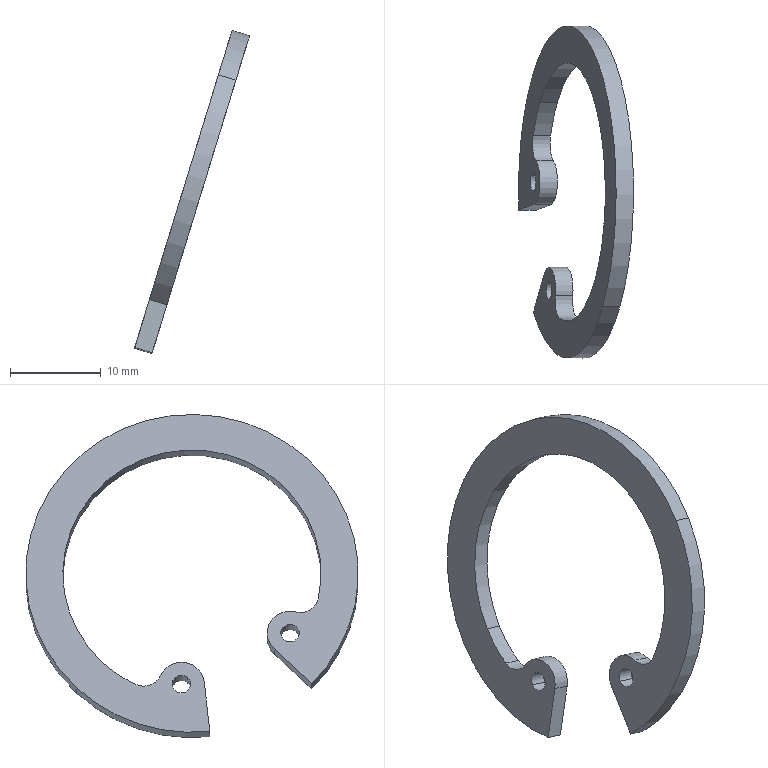Component | SolidWorks | DriveDevice-1_Gasket-2 | 1 solid | 18 faces | box 12.66 x 36.6 x 35.57 mm | volume 802 mm3 | cylinder 14 | plane 4 | commonest cylinder face diameters 2.036 x4 36.6 x3 28.42 x3 4 x2 5.036 x2
build123d program:
from build123d import *

# Parameters (mm, degrees)
SKETCH1_R           = 1.018
BOSS_EXTRUDE1_DEPTH = 2


with BuildPart() as part:
    # Sketch1 → Boss-Extrude1 (new body)
    with BuildSketch(Plane(origin=(0, 0, 0), x_dir=(1, 0, 0), z_dir=(0, 1, 0))):
        with BuildLine():
            Line((14.21, 0), (12.556, 0))
            ThreePointArc((12.556, 0), (10.119, -1.885), (11.331, -4.718))
            ThreePointArc((11.331, -4.718), (12.294, -5.966), (12.054, -7.524))
            ThreePointArc((12.054, -7.524), (-13.353, -4.86), (4.398, 13.512))
            ThreePointArc((4.398, 13.512), (5.583, 12.473), (5.647, 10.898))
            ThreePointArc((5.647, 10.898), (6.54, 7.948), (9.619, 8.071))
            Line((9.619, 8.071), (10.885, 9.134))
            Line((10.885, 9.134), (14.019, 11.763))
            ThreePointArc((14.019, 11.763), (-17.196, -6.259), (18.3, 0))
            Line((18.3, 0), (14.21, 0))
        make_face()
        with Locations(Location((12.556, -2.518, 0), (0, 0, 270))):
            Circle(SKETCH1_R, mode=Mode.SUBTRACT)
        with Locations(Location((8, 10, 0), (0, 0, 270))):
            Circle(SKETCH1_R, mode=Mode.SUBTRACT)
    extrude(amount=BOSS_EXTRUDE1_DEPTH)


solid = part.part

# Placed as in the assembly
solid = solid.moved(Location((-198.473, 15, 12.066), (-95.888, -1.805, 106.985)))
STEP:
#1=COLOUR_RGB('',0.7922,0.8196,0.9333);
#2=FILL_AREA_STYLE_COLOUR('',#1);
#3=FILL_AREA_STYLE('',(#2));
#4=SURFACE_STYLE_FILL_AREA(#3);
#5=SURFACE_SIDE_STYLE('',(#4));
#6=SURFACE_STYLE_USAGE(.BOTH.,#5);
#7=PRESENTATION_STYLE_ASSIGNMENT((#6));
#8=CARTESIAN_POINT('',(-7.885,0.1376,0.2437));
#9=VERTEX_POINT('',#8);
#10=CARTESIAN_POINT('',(-7.902,0.1931,0.1885));
#11=VERTEX_POINT('',#10);
#12=CARTESIAN_POINT('',(-7.893,0.1653,0.2161));
#13=DIRECTION('',(-0.9559,-0.,0.2937));
#14=DIRECTION('',(0.2118,-0.6927,0.6894));
#15=AXIS2_PLACEMENT_3D('',#12,#13,#14);
#16=CIRCLE('',#15,0.04008);
#17=EDGE_CURVE('',#9,#11,#16,.T.);
#18=ORIENTED_EDGE('',*,*,#17,.F.);
#19=CARTESIAN_POINT('',(-7.96,0.1376,0.2668));
#20=VERTEX_POINT('',#19);
#21=CARTESIAN_POINT('',(-7.885,0.1376,0.2437));
#22=DIRECTION('',(-0.9559,-0.,0.2937));
#23=VECTOR('',#22,39.37);
#24=LINE('',#21,#23);
#25=EDGE_CURVE('',#9,#20,#24,.T.);
#26=ORIENTED_EDGE('',*,*,#25,.T.);
#27=CARTESIAN_POINT('',(-7.977,0.1931,0.2116));
#28=VERTEX_POINT('',#27);
#29=CARTESIAN_POINT('',(-7.969,0.1653,0.2392));
#30=DIRECTION('',(-0.9559,-0.,0.2937));
#31=DIRECTION('',(0.2118,-0.6927,0.6894));
#32=AXIS2_PLACEMENT_3D('',#29,#30,#31);
#33=CIRCLE('',#32,0.04008);
#34=EDGE_CURVE('',#20,#28,#33,.T.);
#35=ORIENTED_EDGE('',*,*,#34,.T.);
#36=CARTESIAN_POINT('',(-7.902,0.1931,0.1885));
#37=DIRECTION('',(-0.9559,-0.,0.2937));
#38=VECTOR('',#37,39.37);
#39=LINE('',#36,#38);
#40=EDGE_CURVE('',#11,#28,#39,.T.);
#41=ORIENTED_EDGE('',*,*,#40,.F.);
#42=EDGE_LOOP('',(#18,#26,#35,#41));
#43=FACE_OUTER_BOUND('',#42,.T.);
#44=CARTESIAN_POINT('',(-7.893,0.1653,0.2161));
#45=DIRECTION('',(-0.9559,-0.,0.2937));
#46=DIRECTION('',(-0.2118,0.6927,-0.6894));
#47=AXIS2_PLACEMENT_3D('',#44,#45,#46);
#48=CYLINDRICAL_SURFACE('',#47,0.04008);
#49=ADVANCED_FACE('',(#43),#48,.F.);
#50=CARTESIAN_POINT('',(-7.97,0.6639,-0.03256));
#51=VERTEX_POINT('',#50);
#52=CARTESIAN_POINT('',(-7.953,0.6083,0.02271));
#53=VERTEX_POINT('',#52);
#54=CARTESIAN_POINT('',(-7.961,0.6361,-0.004923));
#55=DIRECTION('',(0.9559,0.,-0.2937));
#56=DIRECTION('',(0.2118,-0.6927,0.6894));
#57=AXIS2_PLACEMENT_3D('',#54,#55,#56);
#58=CIRCLE('',#57,0.04008);
#59=EDGE_CURVE('',#51,#53,#58,.T.);
#60=ORIENTED_EDGE('',*,*,#59,.T.);
#61=CARTESIAN_POINT('',(-8.028,0.6083,0.04584));
#62=VERTEX_POINT('',#61);
#63=CARTESIAN_POINT('',(-7.953,0.6083,0.02271));
#64=DIRECTION('',(-0.9559,-0.,0.2937));
#65=VECTOR('',#64,39.37);
#66=LINE('',#63,#65);
#67=EDGE_CURVE('',#53,#62,#66,.T.);
#68=ORIENTED_EDGE('',*,*,#67,.T.);
#69=CARTESIAN_POINT('',(-8.045,0.6639,-0.009435));
#70=VERTEX_POINT('',#69);
#71=CARTESIAN_POINT('',(-8.037,0.6361,0.0182));
#72=DIRECTION('',(0.9559,0.,-0.2937));
#73=DIRECTION('',(0.2118,-0.6927,0.6894));
#74=AXIS2_PLACEMENT_3D('',#71,#72,#73);
#75=CIRCLE('',#74,0.04008);
#76=EDGE_CURVE('',#70,#62,#75,.T.);
#77=ORIENTED_EDGE('',*,*,#76,.F.);
#78=CARTESIAN_POINT('',(-7.97,0.6639,-0.03256));
#79=DIRECTION('',(-0.9559,-0.,0.2937));
#80=VECTOR('',#79,39.37);
#81=LINE('',#78,#80);
#82=EDGE_CURVE('',#51,#70,#81,.T.);
#83=ORIENTED_EDGE('',*,*,#82,.F.);
#84=EDGE_LOOP('',(#60,#68,#77,#83));
#85=FACE_OUTER_BOUND('',#84,.T.);
#86=CARTESIAN_POINT('',(-7.961,0.6361,-0.004923));
#87=DIRECTION('',(-0.9559,-0.,0.2937));
#88=DIRECTION('',(-0.2118,0.6927,-0.6894));
#89=AXIS2_PLACEMENT_3D('',#86,#87,#88);
#90=CYLINDRICAL_SURFACE('',#89,0.04008);
#91=ADVANCED_FACE('',(#85),#90,.F.);
#92=CARTESIAN_POINT('',(-7.661,0.09149,0.9718));
#93=VERTEX_POINT('',#92);
#94=CARTESIAN_POINT('',(-7.96,0.07092,-0.001994));
#95=VERTEX_POINT('',#94);
#96=CARTESIAN_POINT('',(-7.814,0.5906,0.4751));
#97=DIRECTION('',(0.9559,0.,-0.2937));
#98=DIRECTION('',(0.2118,-0.6927,0.6894));
#99=AXIS2_PLACEMENT_3D('',#96,#97,#98);
#100=CIRCLE('',#99,0.7205);
#101=EDGE_CURVE('',#93,#95,#100,.T.);
#102=ORIENTED_EDGE('',*,*,#101,.F.);
#103=CARTESIAN_POINT('',(-7.737,0.09149,0.9949));
#104=VERTEX_POINT('',#103);
#105=CARTESIAN_POINT('',(-7.661,0.09149,0.9718));
#106=DIRECTION('',(-0.9559,-0.,0.2937));
#107=VECTOR('',#106,39.37);
#108=LINE('',#105,#107);
#109=EDGE_CURVE('',#93,#104,#108,.T.);
#110=ORIENTED_EDGE('',*,*,#109,.T.);
#111=CARTESIAN_POINT('',(-8.036,0.07092,0.02113));
#112=VERTEX_POINT('',#111);
#113=CARTESIAN_POINT('',(-7.889,0.5906,0.4982));
#114=DIRECTION('',(0.9559,0.,-0.2937));
#115=DIRECTION('',(0.2118,-0.6927,0.6894));
#116=AXIS2_PLACEMENT_3D('',#113,#114,#115);
#117=CIRCLE('',#116,0.7205);
#118=EDGE_CURVE('',#104,#112,#117,.T.);
#119=ORIENTED_EDGE('',*,*,#118,.T.);
#120=CARTESIAN_POINT('',(-7.96,0.07092,-0.001994));
#121=DIRECTION('',(-0.9559,-0.,0.2937));
#122=VECTOR('',#121,39.37);
#123=LINE('',#120,#122);
#124=EDGE_CURVE('',#95,#112,#123,.T.);
#125=ORIENTED_EDGE('',*,*,#124,.F.);
#126=EDGE_LOOP('',(#102,#110,#119,#125));
#127=FACE_OUTER_BOUND('',#126,.T.);
#128=CARTESIAN_POINT('',(-7.814,0.5906,0.4751));
#129=DIRECTION('',(-0.9559,-0.,0.2937));
#130=DIRECTION('',(-0.2118,0.6927,-0.6894));
#131=AXIS2_PLACEMENT_3D('',#128,#129,#130);
#132=CYLINDRICAL_SURFACE('',#131,0.7205);
#133=ADVANCED_FACE('',(#127),#132,.T.);
#134=ORIENTED_EDGE('',*,*,#109,.F.);
#135=CARTESIAN_POINT('',(-7.967,1.09,-0.02167));
#136=VERTEX_POINT('',#135);
#137=CARTESIAN_POINT('',(-7.814,0.5906,0.4751));
#138=DIRECTION('',(0.9559,0.,-0.2937));
#139=DIRECTION('',(0.2118,-0.6927,0.6894));
#140=AXIS2_PLACEMENT_3D('',#137,#138,#139);
#141=CIRCLE('',#140,0.7205);
#142=EDGE_CURVE('',#136,#93,#141,.T.);
#143=ORIENTED_EDGE('',*,*,#142,.F.);
#144=CARTESIAN_POINT('',(-8.042,1.09,0.001459));
#145=VERTEX_POINT('',#144);
#146=CARTESIAN_POINT('',(-7.967,1.09,-0.02167));
#147=DIRECTION('',(-0.9559,-0.,0.2937));
#148=VECTOR('',#147,39.37);
#149=LINE('',#146,#148);
#150=EDGE_CURVE('',#136,#145,#149,.T.);
#151=ORIENTED_EDGE('',*,*,#150,.T.);
#152=CARTESIAN_POINT('',(-7.889,0.5906,0.4982));
#153=DIRECTION('',(0.9559,0.,-0.2937));
#154=DIRECTION('',(0.2118,-0.6927,0.6894));
#155=AXIS2_PLACEMENT_3D('',#152,#153,#154);
#156=CIRCLE('',#155,0.7205);
#157=EDGE_CURVE('',#145,#104,#156,.T.);
#158=ORIENTED_EDGE('',*,*,#157,.T.);
#159=EDGE_LOOP('',(#134,#143,#151,#158));
#160=FACE_OUTER_BOUND('',#159,.T.);
#161=CARTESIAN_POINT('',(-7.814,0.5906,0.4751));
#162=DIRECTION('',(-0.9559,-0.,0.2937));
#163=DIRECTION('',(-0.2118,0.6927,-0.6894));
#164=AXIS2_PLACEMENT_3D('',#161,#162,#163);
#165=CYLINDRICAL_SURFACE('',#164,0.7205);
#166=ADVANCED_FACE('',(#160),#165,.T.);
#167=CARTESIAN_POINT('',(-7.932,0.9781,0.08935));
#168=VERTEX_POINT('',#167);
#169=CARTESIAN_POINT('',(-7.695,0.203,0.8608));
#170=VERTEX_POINT('',#169);
#171=CARTESIAN_POINT('',(-7.814,0.5906,0.4751));
#172=DIRECTION('',(0.9559,0.,-0.2937));
#173=DIRECTION('',(0.2118,-0.6927,0.6894));
#174=AXIS2_PLACEMENT_3D('',#171,#172,#173);
#175=CIRCLE('',#174,0.5594);
#176=EDGE_CURVE('',#168,#170,#175,.T.);
#177=ORIENTED_EDGE('',*,*,#176,.T.);
#178=CARTESIAN_POINT('',(-7.771,0.203,0.8839));
#179=VERTEX_POINT('',#178);
#180=CARTESIAN_POINT('',(-7.695,0.203,0.8608));
#181=DIRECTION('',(-0.9559,-0.,0.2937));
#182=VECTOR('',#181,39.37);
#183=LINE('',#180,#182);
#184=EDGE_CURVE('',#170,#179,#183,.T.);
#185=ORIENTED_EDGE('',*,*,#184,.T.);
#186=CARTESIAN_POINT('',(-8.008,0.9781,0.1125));
#187=VERTEX_POINT('',#186);
#188=CARTESIAN_POINT('',(-7.889,0.5906,0.4982));
#189=DIRECTION('',(0.9559,0.,-0.2937));
#190=DIRECTION('',(0.2118,-0.6927,0.6894));
#191=AXIS2_PLACEMENT_3D('',#188,#189,#190);
#192=CIRCLE('',#191,0.5594);
#193=EDGE_CURVE('',#187,#179,#192,.T.);
#194=ORIENTED_EDGE('',*,*,#193,.F.);
#195=CARTESIAN_POINT('',(-7.932,0.9781,0.08935));
#196=DIRECTION('',(-0.9559,-0.,0.2937));
#197=VECTOR('',#196,39.37);
#198=LINE('',#195,#197);
#199=EDGE_CURVE('',#168,#187,#198,.T.);
#200=ORIENTED_EDGE('',*,*,#199,.F.);
#201=EDGE_LOOP('',(#177,#185,#194,#200));
#202=FACE_OUTER_BOUND('',#201,.T.);
#203=CARTESIAN_POINT('',(-7.814,0.5906,0.4751));
#204=DIRECTION('',(-0.9559,-0.,0.2937));
#205=DIRECTION('',(-0.2118,0.6927,-0.6894));
#206=AXIS2_PLACEMENT_3D('',#203,#204,#205);
#207=CYLINDRICAL_SURFACE('',#206,0.5594);
#208=ADVANCED_FACE('',(#202),#207,.F.);
#209=CARTESIAN_POINT('',(-7.962,0.8342,-0.006353));
#210=VERTEX_POINT('',#209);
#211=CARTESIAN_POINT('',(-7.814,0.5906,0.4751));
#212=DIRECTION('',(0.9559,0.,-0.2937));
#213=DIRECTION('',(0.2118,-0.6927,0.6894));
#214=AXIS2_PLACEMENT_3D('',#211,#212,#213);
#215=CIRCLE('',#214,0.5594);
#216=EDGE_CURVE('',#210,#168,#215,.T.);
#217=ORIENTED_EDGE('',*,*,#216,.T.);
#218=ORIENTED_EDGE('',*,*,#199,.T.);
#219=CARTESIAN_POINT('',(-8.037,0.8342,0.01677));
#220=VERTEX_POINT('',#219);
#221=CARTESIAN_POINT('',(-7.889,0.5906,0.4982));
#222=DIRECTION('',(0.9559,0.,-0.2937));
#223=DIRECTION('',(0.2118,-0.6927,0.6894));
#224=AXIS2_PLACEMENT_3D('',#221,#222,#223);
#225=CIRCLE('',#224,0.5594);
#226=EDGE_CURVE('',#220,#187,#225,.T.);
#227=ORIENTED_EDGE('',*,*,#226,.F.);
#228=CARTESIAN_POINT('',(-7.962,0.8342,-0.006353));
#229=DIRECTION('',(-0.9559,-0.,0.2937));
#230=VECTOR('',#229,39.37);
#231=LINE('',#228,#230);
#232=EDGE_CURVE('',#210,#220,#231,.T.);
#233=ORIENTED_EDGE('',*,*,#232,.F.);
#234=EDGE_LOOP('',(#217,#218,#227,#233));
#235=FACE_OUTER_BOUND('',#234,.T.);
#236=CARTESIAN_POINT('',(-7.814,0.5906,0.4751));
#237=DIRECTION('',(-0.9559,-0.,0.2937));
#238=DIRECTION('',(-0.2118,0.6927,-0.6894));
#239=AXIS2_PLACEMENT_3D('',#236,#237,#238);
#240=CYLINDRICAL_SURFACE('',#239,0.5594);
#241=ADVANCED_FACE('',(#235),#240,.F.);
#242=CARTESIAN_POINT('',(-7.923,0.04307,0.3882));
#243=VERTEX_POINT('',#242);
#244=CARTESIAN_POINT('',(-7.941,0.1401,0.3309));
#245=VERTEX_POINT('',#244);
#246=CARTESIAN_POINT('',(-7.918,0.1201,0.4037));
#247=DIRECTION('',(0.9559,0.,-0.2937));
#248=DIRECTION('',(0.2118,-0.6927,0.6894));
#249=AXIS2_PLACEMENT_3D('',#246,#247,#248);
#250=CIRCLE('',#249,0.07874);
#251=EDGE_CURVE('',#243,#245,#250,.T.);
#252=ORIENTED_EDGE('',*,*,#251,.F.);
#253=CARTESIAN_POINT('',(-7.848,0.04307,0.3651));
#254=VERTEX_POINT('',#253);
#255=CARTESIAN_POINT('',(-7.848,0.04307,0.3651));
#256=DIRECTION('',(-0.9559,-0.,0.2937));
#257=VECTOR('',#256,39.37);
#258=LINE('',#255,#257);
#259=EDGE_CURVE('',#254,#243,#258,.T.);
#260=ORIENTED_EDGE('',*,*,#259,.F.);
#261=CARTESIAN_POINT('',(-7.865,0.1401,0.3077));
#262=VERTEX_POINT('',#261);
#263=CARTESIAN_POINT('',(-7.843,0.1201,0.3805));
#264=DIRECTION('',(0.9559,0.,-0.2937));
#265=DIRECTION('',(0.2118,-0.6927,0.6894));
#266=AXIS2_PLACEMENT_3D('',#263,#264,#265);
#267=CIRCLE('',#266,0.07874);
#268=EDGE_CURVE('',#254,#262,#267,.T.);
#269=ORIENTED_EDGE('',*,*,#268,.T.);
#270=CARTESIAN_POINT('',(-7.865,0.1401,0.3077));
#271=DIRECTION('',(-0.9559,-0.,0.2937));
#272=VECTOR('',#271,39.37);
#273=LINE('',#270,#272);
#274=EDGE_CURVE('',#262,#245,#273,.T.);
#275=ORIENTED_EDGE('',*,*,#274,.T.);
#276=EDGE_LOOP('',(#252,#260,#269,#275));
#277=FACE_OUTER_BOUND('',#276,.T.);
#278=CARTESIAN_POINT('',(-7.843,0.1201,0.3805));
#279=DIRECTION('',(-0.9559,-0.,0.2937));
#280=DIRECTION('',(-0.2118,0.6927,-0.6894));
#281=AXIS2_PLACEMENT_3D('',#278,#279,#280);
#282=CYLINDRICAL_SURFACE('',#281,0.07874);
#283=ADVANCED_FACE('',(#277),#282,.F.);
#284=ORIENTED_EDGE('',*,*,#184,.F.);
#285=CARTESIAN_POINT('',(-7.814,0.5906,0.4751));
#286=DIRECTION('',(0.9559,0.,-0.2937));
#287=DIRECTION('',(0.2118,-0.6927,0.6894));
#288=AXIS2_PLACEMENT_3D('',#285,#286,#287);
#289=CIRCLE('',#288,0.5594);
#290=EDGE_CURVE('',#170,#254,#289,.T.);
#291=ORIENTED_EDGE('',*,*,#290,.T.);
#292=ORIENTED_EDGE('',*,*,#259,.T.);
#293=CARTESIAN_POINT('',(-7.889,0.5906,0.4982));
#294=DIRECTION('',(0.9559,0.,-0.2937));
#295=DIRECTION('',(0.2118,-0.6927,0.6894));
#296=AXIS2_PLACEMENT_3D('',#293,#294,#295);
#297=CIRCLE('',#296,0.5594);
#298=EDGE_CURVE('',#179,#243,#297,.T.);
#299=ORIENTED_EDGE('',*,*,#298,.F.);
#300=EDGE_LOOP('',(#284,#291,#292,#299));
#301=FACE_OUTER_BOUND('',#300,.T.);
#302=CARTESIAN_POINT('',(-7.814,0.5906,0.4751));
#303=DIRECTION('',(-0.9559,-0.,0.2937));
#304=DIRECTION('',(-0.2118,0.6927,-0.6894));
#305=AXIS2_PLACEMENT_3D('',#302,#303,#304);
#306=CYLINDRICAL_SURFACE('',#305,0.5594);
#307=ADVANCED_FACE('',(#301),#306,.F.);
#308=CARTESIAN_POINT('',(-8.025,0.7274,0.05517));
#309=VERTEX_POINT('',#308);
#310=CARTESIAN_POINT('',(-8.016,0.7999,0.08453));
#311=DIRECTION('',(-0.9559,-0.,0.2937));
#312=DIRECTION('',(0.2118,-0.6927,0.6894));
#313=AXIS2_PLACEMENT_3D('',#310,#311,#312);
#314=CIRCLE('',#313,0.07874);
#315=EDGE_CURVE('',#220,#309,#314,.T.);
#316=ORIENTED_EDGE('',*,*,#315,.T.);
#317=CARTESIAN_POINT('',(-7.95,0.7274,0.03204));
#318=VERTEX_POINT('',#317);
#319=CARTESIAN_POINT('',(-7.95,0.7274,0.03204));
#320=DIRECTION('',(-0.9559,-0.,0.2937));
#321=VECTOR('',#320,39.37);
#322=LINE('',#319,#321);
#323=EDGE_CURVE('',#318,#309,#322,.T.);
#324=ORIENTED_EDGE('',*,*,#323,.F.);
#325=CARTESIAN_POINT('',(-7.941,0.7999,0.0614));
#326=DIRECTION('',(-0.9559,-0.,0.2937));
#327=DIRECTION('',(0.2118,-0.6927,0.6894));
#328=AXIS2_PLACEMENT_3D('',#325,#326,#327);
#329=CIRCLE('',#328,0.07874);
#330=EDGE_CURVE('',#210,#318,#329,.T.);
#331=ORIENTED_EDGE('',*,*,#330,.F.);
#332=ORIENTED_EDGE('',*,*,#232,.T.);
#333=EDGE_LOOP('',(#316,#324,#331,#332));
#334=FACE_OUTER_BOUND('',#333,.T.);
#335=CARTESIAN_POINT('',(-7.941,0.7999,0.0614));
#336=DIRECTION('',(-0.9559,-0.,0.2937));
#337=DIRECTION('',(-0.2118,0.6927,-0.6894));
#338=AXIS2_PLACEMENT_3D('',#335,#336,#337);
#339=CYLINDRICAL_SURFACE('',#338,0.07874);
#340=ADVANCED_FACE('',(#334),#339,.F.);
#341=CARTESIAN_POINT('',(-8.034,0.5375,0.02837));
#342=VERTEX_POINT('',#341);
#343=CARTESIAN_POINT('',(-8.037,0.6361,0.0182));
#344=DIRECTION('',(0.9559,0.,-0.2937));
#345=DIRECTION('',(0.2118,-0.6927,0.6894));
#346=AXIS2_PLACEMENT_3D('',#343,#344,#345);
#347=CIRCLE('',#346,0.09914);
#348=EDGE_CURVE('',#309,#342,#347,.T.);
#349=ORIENTED_EDGE('',*,*,#348,.T.);
#350=CARTESIAN_POINT('',(-7.958,0.5375,0.005242));
#351=VERTEX_POINT('',#350);
#352=CARTESIAN_POINT('',(-7.958,0.5375,0.005242));
#353=DIRECTION('',(-0.9559,-0.,0.2937));
#354=VECTOR('',#353,39.37);
#355=LINE('',#352,#354);
#356=EDGE_CURVE('',#351,#342,#355,.T.);
#357=ORIENTED_EDGE('',*,*,#356,.F.);
#358=CARTESIAN_POINT('',(-7.961,0.6361,-0.004923));
#359=DIRECTION('',(0.9559,0.,-0.2937));
#360=DIRECTION('',(0.2118,-0.6927,0.6894));
#361=AXIS2_PLACEMENT_3D('',#358,#359,#360);
#362=CIRCLE('',#361,0.09914);
#363=EDGE_CURVE('',#318,#351,#362,.T.);
#364=ORIENTED_EDGE('',*,*,#363,.F.);
#365=ORIENTED_EDGE('',*,*,#323,.T.);
#366=EDGE_LOOP('',(#349,#357,#364,#365));
#367=FACE_OUTER_BOUND('',#366,.T.);
#368=CARTESIAN_POINT('',(-7.961,0.6361,-0.004923));
#369=DIRECTION('',(-0.9559,-0.,0.2937));
#370=DIRECTION('',(-0.2118,0.6927,-0.6894));
#371=AXIS2_PLACEMENT_3D('',#368,#369,#370);
#372=CYLINDRICAL_SURFACE('',#371,0.09914);
#373=ADVANCED_FACE('',(#367),#372,.T.);
#374=CARTESIAN_POINT('',(-8.1,0.5133,-0.1865));
#375=VERTEX_POINT('',#374);
#376=CARTESIAN_POINT('',(-7.889,0.5906,0.4982));
#377=DIRECTION('',(-0.292,-0.1073,-0.9504));
#378=VECTOR('',#377,39.37);
#379=LINE('',#376,#378);
#380=EDGE_CURVE('',#342,#375,#379,.T.);
#381=ORIENTED_EDGE('',*,*,#380,.T.);
#382=CARTESIAN_POINT('',(-8.024,0.5133,-0.2097));
#383=VERTEX_POINT('',#382);
#384=CARTESIAN_POINT('',(-8.024,0.5133,-0.2097));
#385=DIRECTION('',(-0.9559,-0.,0.2937));
#386=VECTOR('',#385,39.37);
#387=LINE('',#384,#386);
#388=EDGE_CURVE('',#383,#375,#387,.T.);
#389=ORIENTED_EDGE('',*,*,#388,.F.);
#390=CARTESIAN_POINT('',(-7.814,0.5906,0.4751));
#391=DIRECTION('',(-0.292,-0.1073,-0.9504));
#392=VECTOR('',#391,39.37);
#393=LINE('',#390,#392);
#394=EDGE_CURVE('',#351,#383,#393,.T.);
#395=ORIENTED_EDGE('',*,*,#394,.F.);
#396=ORIENTED_EDGE('',*,*,#356,.T.);
#397=EDGE_LOOP('',(#381,#389,#395,#396));
#398=FACE_OUTER_BOUND('',#397,.T.);
#399=CARTESIAN_POINT('',(-7.814,0.5906,0.4751));
#400=DIRECTION('',(-0.0315,0.9942,-0.1025));
#401=DIRECTION('',(0.292,0.1073,0.9504));
#402=AXIS2_PLACEMENT_3D('',#399,#400,#401);
#403=PLANE('',#402);
#404=ADVANCED_FACE('',(#398),#403,.F.);
#405=ORIENTED_EDGE('',*,*,#150,.F.);
#406=CARTESIAN_POINT('',(-7.814,0.5906,0.4751));
#407=DIRECTION('',(0.9559,0.,-0.2937));
#408=DIRECTION('',(0.2118,-0.6927,0.6894));
#409=AXIS2_PLACEMENT_3D('',#406,#407,#408);
#410=CIRCLE('',#409,0.7205);
#411=EDGE_CURVE('',#383,#136,#410,.T.);
#412=ORIENTED_EDGE('',*,*,#411,.F.);
#413=ORIENTED_EDGE('',*,*,#388,.T.);
#414=CARTESIAN_POINT('',(-7.889,0.5906,0.4982));
#415=DIRECTION('',(0.9559,0.,-0.2937));
#416=DIRECTION('',(0.2118,-0.6927,0.6894));
#417=AXIS2_PLACEMENT_3D('',#414,#415,#416);
#418=CIRCLE('',#417,0.7205);
#419=EDGE_CURVE('',#375,#145,#418,.T.);
#420=ORIENTED_EDGE('',*,*,#419,.T.);
#421=EDGE_LOOP('',(#405,#412,#413,#420));
#422=FACE_OUTER_BOUND('',#421,.T.);
#423=CARTESIAN_POINT('',(-7.814,0.5906,0.4751));
#424=DIRECTION('',(-0.9559,-0.,0.2937));
#425=DIRECTION('',(-0.2118,0.6927,-0.6894));
#426=AXIS2_PLACEMENT_3D('',#423,#424,#425);
#427=CYLINDRICAL_SURFACE('',#426,0.7205);
#428=ADVANCED_FACE('',(#422),#427,.T.);
#429=CARTESIAN_POINT('',(-7.99,0.234,0.1709));
#430=VERTEX_POINT('',#429);
#431=CARTESIAN_POINT('',(-7.889,0.5906,0.4982));
#432=DIRECTION('',(-0.2034,-0.7212,-0.6621));
#433=VECTOR('',#432,39.37);
#434=LINE('',#431,#433);
#435=EDGE_CURVE('',#430,#112,#434,.T.);
#436=ORIENTED_EDGE('',*,*,#435,.F.);
#437=CARTESIAN_POINT('',(-7.914,0.234,0.1477));
#438=VERTEX_POINT('',#437);
#439=CARTESIAN_POINT('',(-7.914,0.234,0.1477));
#440=DIRECTION('',(-0.9559,-0.,0.2937));
#441=VECTOR('',#440,39.37);
#442=LINE('',#439,#441);
#443=EDGE_CURVE('',#438,#430,#442,.T.);
#444=ORIENTED_EDGE('',*,*,#443,.F.);
#445=CARTESIAN_POINT('',(-7.814,0.5906,0.4751));
#446=DIRECTION('',(-0.2034,-0.7212,-0.6621));
#447=VECTOR('',#446,39.37);
#448=LINE('',#445,#447);
#449=EDGE_CURVE('',#438,#95,#448,.T.);
#450=ORIENTED_EDGE('',*,*,#449,.T.);
#451=ORIENTED_EDGE('',*,*,#124,.T.);
#452=EDGE_LOOP('',(#436,#444,#450,#451));
#453=FACE_OUTER_BOUND('',#452,.T.);
#454=CARTESIAN_POINT('',(-7.814,0.5906,0.4751));
#455=DIRECTION('',(-0.2118,0.6927,-0.6894));
#456=DIRECTION('',(0.2034,0.7212,0.6621));
#457=AXIS2_PLACEMENT_3D('',#454,#455,#456);
#458=PLANE('',#457);
#459=ADVANCED_FACE('',(#453),#458,.T.);
#460=ORIENTED_EDGE('',*,*,#67,.F.);
#461=CARTESIAN_POINT('',(-7.961,0.6361,-0.004923));
#462=DIRECTION('',(0.9559,0.,-0.2937));
#463=DIRECTION('',(0.2118,-0.6927,0.6894));
#464=AXIS2_PLACEMENT_3D('',#461,#462,#463);
#465=CIRCLE('',#464,0.04008);
#466=EDGE_CURVE('',#53,#51,#465,.T.);
#467=ORIENTED_EDGE('',*,*,#466,.T.);
#468=ORIENTED_EDGE('',*,*,#82,.T.);
#469=CARTESIAN_POINT('',(-8.037,0.6361,0.0182));
#470=DIRECTION('',(0.9559,0.,-0.2937));
#471=DIRECTION('',(0.2118,-0.6927,0.6894));
#472=AXIS2_PLACEMENT_3D('',#469,#470,#471);
#473=CIRCLE('',#472,0.04008);
#474=EDGE_CURVE('',#62,#70,#473,.T.);
#475=ORIENTED_EDGE('',*,*,#474,.F.);
#476=EDGE_LOOP('',(#460,#467,#468,#475));
#477=FACE_OUTER_BOUND('',#476,.T.);
#478=CARTESIAN_POINT('',(-7.961,0.6361,-0.004923));
#479=DIRECTION('',(-0.9559,-0.,0.2937));
#480=DIRECTION('',(-0.2118,0.6927,-0.6894));
#481=AXIS2_PLACEMENT_3D('',#478,#479,#480);
#482=CYLINDRICAL_SURFACE('',#481,0.04008);
#483=ADVANCED_FACE('',(#477),#482,.F.);
#484=CARTESIAN_POINT('',(-7.969,0.1653,0.2392));
#485=DIRECTION('',(-0.9559,-0.,0.2937));
#486=DIRECTION('',(0.2118,-0.6927,0.6894));
#487=AXIS2_PLACEMENT_3D('',#484,#485,#486);
#488=CIRCLE('',#487,0.09914);
#489=EDGE_CURVE('',#245,#430,#488,.T.);
#490=ORIENTED_EDGE('',*,*,#489,.F.);
#491=ORIENTED_EDGE('',*,*,#274,.F.);
#492=CARTESIAN_POINT('',(-7.893,0.1653,0.2161));
#493=DIRECTION('',(-0.9559,-0.,0.2937));
#494=DIRECTION('',(0.2118,-0.6927,0.6894));
#495=AXIS2_PLACEMENT_3D('',#492,#493,#494);
#496=CIRCLE('',#495,0.09914);
#497=EDGE_CURVE('',#262,#438,#496,.T.);
#498=ORIENTED_EDGE('',*,*,#497,.T.);
#499=ORIENTED_EDGE('',*,*,#443,.T.);
#500=EDGE_LOOP('',(#490,#491,#498,#499));
#501=FACE_OUTER_BOUND('',#500,.T.);
#502=CARTESIAN_POINT('',(-7.893,0.1653,0.2161));
#503=DIRECTION('',(-0.9559,-0.,0.2937));
#504=DIRECTION('',(-0.2118,0.6927,-0.6894));
#505=AXIS2_PLACEMENT_3D('',#502,#503,#504);
#506=CYLINDRICAL_SURFACE('',#505,0.09914);
#507=ADVANCED_FACE('',(#501),#506,.T.);
#508=ORIENTED_EDGE('',*,*,#25,.F.);
#509=CARTESIAN_POINT('',(-7.893,0.1653,0.2161));
#510=DIRECTION('',(-0.9559,-0.,0.2937));
#511=DIRECTION('',(0.2118,-0.6927,0.6894));
#512=AXIS2_PLACEMENT_3D('',#509,#510,#511);
#513=CIRCLE('',#512,0.04008);
#514=EDGE_CURVE('',#11,#9,#513,.T.);
#515=ORIENTED_EDGE('',*,*,#514,.F.);
#516=ORIENTED_EDGE('',*,*,#40,.T.);
#517=CARTESIAN_POINT('',(-7.969,0.1653,0.2392));
#518=DIRECTION('',(-0.9559,-0.,0.2937));
#519=DIRECTION('',(0.2118,-0.6927,0.6894));
#520=AXIS2_PLACEMENT_3D('',#517,#518,#519);
#521=CIRCLE('',#520,0.04008);
#522=EDGE_CURVE('',#28,#20,#521,.T.);
#523=ORIENTED_EDGE('',*,*,#522,.T.);
#524=EDGE_LOOP('',(#508,#515,#516,#523));
#525=FACE_OUTER_BOUND('',#524,.T.);
#526=CARTESIAN_POINT('',(-7.893,0.1653,0.2161));
#527=DIRECTION('',(-0.9559,-0.,0.2937));
#528=DIRECTION('',(-0.2118,0.6927,-0.6894));
#529=AXIS2_PLACEMENT_3D('',#526,#527,#528);
#530=CYLINDRICAL_SURFACE('',#529,0.04008);
#531=ADVANCED_FACE('',(#525),#530,.F.);
#532=ORIENTED_EDGE('',*,*,#268,.F.);
#533=ORIENTED_EDGE('',*,*,#290,.F.);
#534=ORIENTED_EDGE('',*,*,#176,.F.);
#535=ORIENTED_EDGE('',*,*,#216,.F.);
#536=ORIENTED_EDGE('',*,*,#330,.T.);
#537=ORIENTED_EDGE('',*,*,#363,.T.);
#538=ORIENTED_EDGE('',*,*,#394,.T.);
#539=ORIENTED_EDGE('',*,*,#411,.T.);
#540=ORIENTED_EDGE('',*,*,#142,.T.);
#541=ORIENTED_EDGE('',*,*,#101,.T.);
#542=ORIENTED_EDGE('',*,*,#449,.F.);
#543=ORIENTED_EDGE('',*,*,#497,.F.);
#544=EDGE_LOOP('',(#532,#533,#534,#535,#536,#537,#538,#539,#540,#541,#542,#543));
#545=FACE_OUTER_BOUND('',#544,.T.);
#546=ORIENTED_EDGE('',*,*,#59,.F.);
#547=ORIENTED_EDGE('',*,*,#466,.F.);
#548=EDGE_LOOP('',(#546,#547));
#549=FACE_BOUND('',#548,.T.);
#550=ORIENTED_EDGE('',*,*,#514,.T.);
#551=ORIENTED_EDGE('',*,*,#17,.T.);
#552=EDGE_LOOP('',(#550,#551));
#553=FACE_BOUND('',#552,.T.);
#554=CARTESIAN_POINT('',(-7.814,0.5906,0.4751));
#555=DIRECTION('',(0.9559,0.,-0.2937));
#556=DIRECTION('',(0.2118,-0.6927,0.6894));
#557=AXIS2_PLACEMENT_3D('',#554,#555,#556);
#558=PLANE('',#557);
#559=ADVANCED_FACE('',(#545,#549,#553),#558,.T.);
#560=ORIENTED_EDGE('',*,*,#251,.T.);
#561=ORIENTED_EDGE('',*,*,#489,.T.);
#562=ORIENTED_EDGE('',*,*,#435,.T.);
#563=ORIENTED_EDGE('',*,*,#118,.F.);
#564=ORIENTED_EDGE('',*,*,#157,.F.);
#565=ORIENTED_EDGE('',*,*,#419,.F.);
#566=ORIENTED_EDGE('',*,*,#380,.F.);
#567=ORIENTED_EDGE('',*,*,#348,.F.);
#568=ORIENTED_EDGE('',*,*,#315,.F.);
#569=ORIENTED_EDGE('',*,*,#226,.T.);
#570=ORIENTED_EDGE('',*,*,#193,.T.);
#571=ORIENTED_EDGE('',*,*,#298,.T.);
#572=EDGE_LOOP('',(#560,#561,#562,#563,#564,#565,#566,#567,#568,#569,#570,#571));
#573=FACE_OUTER_BOUND('',#572,.T.);
#574=ORIENTED_EDGE('',*,*,#76,.T.);
#575=ORIENTED_EDGE('',*,*,#474,.T.);
#576=EDGE_LOOP('',(#574,#575));
#577=FACE_BOUND('',#576,.T.);
#578=ORIENTED_EDGE('',*,*,#522,.F.);
#579=ORIENTED_EDGE('',*,*,#34,.F.);
#580=EDGE_LOOP('',(#578,#579));
#581=FACE_BOUND('',#580,.T.);
#582=CARTESIAN_POINT('',(-7.889,0.5906,0.4982));
#583=DIRECTION('',(0.9559,0.,-0.2937));
#584=DIRECTION('',(0.2118,-0.6927,0.6894));
#585=AXIS2_PLACEMENT_3D('',#582,#583,#584);
#586=PLANE('',#585);
#587=ADVANCED_FACE('',(#573,#577,#581),#586,.F.);
#588=CLOSED_SHELL('',(#49,#91,#133,#166,#208,#241,#283,#307,#340,#373,#404,#428,#459,#483,#507,#531,#559,#587));
#589=MANIFOLD_SOLID_BREP('',#588);
#590=STYLED_ITEM('',(#7),#589);
#591=PRESENTATION_LAYER_ASSIGNMENT('','',(#590));
#592=(LENGTH_UNIT()NAMED_UNIT(*)SI_UNIT($,.METRE.));
#593=LENGTH_MEASURE_WITH_UNIT(LENGTH_MEASURE(0.0254),#592);
#594=DIMENSIONAL_EXPONENTS(1.,0.,0.,0.,0.,0.,0.);
#595=(CONVERSION_BASED_UNIT('',#593)LENGTH_UNIT()NAMED_UNIT(#594));
#596=UNCERTAINTY_MEASURE_WITH_UNIT(LENGTH_MEASURE(0.00001),#595,'','');
#597=(NAMED_UNIT(*)PLANE_ANGLE_UNIT()SI_UNIT($,.RADIAN.));
#598=(NAMED_UNIT(*)SI_UNIT($,.STERADIAN.)SOLID_ANGLE_UNIT());
#599=(GEOMETRIC_REPRESENTATION_CONTEXT(3)GLOBAL_UNCERTAINTY_ASSIGNED_CONTEXT((#596))GLOBAL_UNIT_ASSIGNED_CONTEXT((#595,#597,#598))REPRESENTATION_CONTEXT('',''));
#600=MECHANICAL_DESIGN_GEOMETRIC_PRESENTATION_REPRESENTATION('',(#590),#599);
#601=CARTESIAN_POINT('',(0.,0.,0.));
#602=DIRECTION('',(0.,0.,1.));
#603=DIRECTION('',(1.,0.,0.));
#604=AXIS2_PLACEMENT_3D('',#601,#602,#603);
#605=(LENGTH_UNIT()NAMED_UNIT(*)SI_UNIT($,.METRE.));
#606=LENGTH_MEASURE_WITH_UNIT(LENGTH_MEASURE(0.0254),#605);
#607=DIMENSIONAL_EXPONENTS(1.,0.,0.,0.,0.,0.,0.);
#608=(CONVERSION_BASED_UNIT('',#606)LENGTH_UNIT()NAMED_UNIT(#607));
#609=UNCERTAINTY_MEASURE_WITH_UNIT(LENGTH_MEASURE(0.00001),#608,'','');
#610=(NAMED_UNIT(*)PLANE_ANGLE_UNIT()SI_UNIT($,.RADIAN.));
#611=(NAMED_UNIT(*)SI_UNIT($,.STERADIAN.)SOLID_ANGLE_UNIT());
#612=(GEOMETRIC_REPRESENTATION_CONTEXT(3)GLOBAL_UNCERTAINTY_ASSIGNED_CONTEXT((#609))GLOBAL_UNIT_ASSIGNED_CONTEXT((#608,#610,#611))REPRESENTATION_CONTEXT('',''));
#613=ADVANCED_BREP_SHAPE_REPRESENTATION('',(#589,#604),#612);